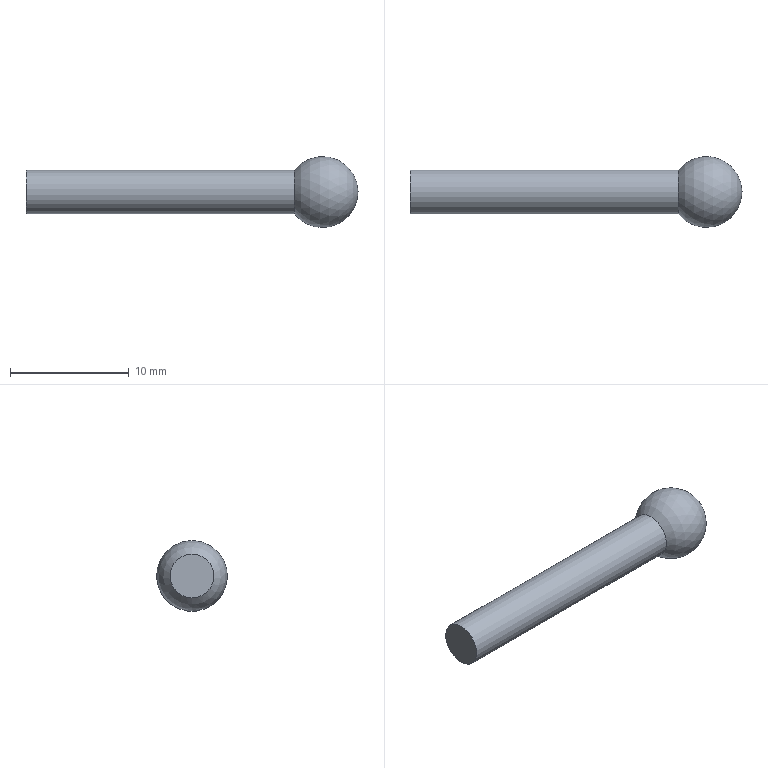Component | NX | CONE_VALVE | 1 solid | 3 faces | box 28 x 6 x 6 mm | volume 353 mm3 | sphere 1 | cylinder 1 | plane 1 | commonest cylinder face diameters 3.7 x1
STEP:
#1=CARTESIAN_POINT('',(0.,0.,0.));
#2=DIRECTION('',(0.,0.,1.));
#3=DIRECTION('',(1.,0.,0.));
#4=AXIS2_PLACEMENT_3D('',#1,#2,#3);
#5=CARTESIAN_POINT('',(-0.5,-0.,18.15));
#6=VERTEX_POINT('',#5);
#7=CARTESIAN_POINT('',(-0.5,-0.,20.));
#8=DIRECTION('',(-1.,0.,0.));
#9=DIRECTION('',(0.,0.,-1.));
#10=AXIS2_PLACEMENT_3D('',#7,#8,#9);
#11=CIRCLE('',#10,1.85);
#12=CARTESIAN_POINT('',(1.862,-0.,20.));
#13=DIRECTION('',(1.,0.,0.));
#14=DIRECTION('',(0.,0.,-1.));
#15=AXIS2_PLACEMENT_3D('',#12,#13,#14);
#16=SPHERICAL_SURFACE('',#15,3.);
#17=CARTESIAN_POINT('',(6.283,-0.9063));
#18=CARTESIAN_POINT('',(6.188,-0.9063));
#19=CARTESIAN_POINT('',(5.998,-0.9063));
#20=CARTESIAN_POINT('',(5.712,-0.9063));
#21=CARTESIAN_POINT('',(5.426,-0.9063));
#22=CARTESIAN_POINT('',(5.141,-0.9063));
#23=CARTESIAN_POINT('',(4.855,-0.9063));
#24=CARTESIAN_POINT('',(4.57,-0.9063));
#25=CARTESIAN_POINT('',(4.284,-0.9063));
#26=CARTESIAN_POINT('',(3.998,-0.9063));
#27=CARTESIAN_POINT('',(3.713,-0.9063));
#28=CARTESIAN_POINT('',(3.427,-0.9063));
#29=CARTESIAN_POINT('',(3.142,-0.9063));
#30=CARTESIAN_POINT('',(2.856,-0.9063));
#31=CARTESIAN_POINT('',(2.57,-0.9063));
#32=CARTESIAN_POINT('',(2.285,-0.9063));
#33=CARTESIAN_POINT('',(1.999,-0.9063));
#34=CARTESIAN_POINT('',(1.714,-0.9063));
#35=CARTESIAN_POINT('',(1.428,-0.9063));
#36=CARTESIAN_POINT('',(1.142,-0.9063));
#37=CARTESIAN_POINT('',(0.8568,-0.9063));
#38=CARTESIAN_POINT('',(0.5712,-0.9063));
#39=CARTESIAN_POINT('',(0.2856,-0.9063));
#40=CARTESIAN_POINT('',(0.0952,-0.9063));
#41=CARTESIAN_POINT('',(0.,-0.9063));
#42=B_SPLINE_CURVE_WITH_KNOTS('',3,(#17,#18,#19,#20,#21,#22,#23,#24,#25,#26,#27,#28,#29,#30,#31,#32,#33,#34,#35,#36,#37,#38,#39,#40,#41),.UNSPECIFIED.,.F.,.F.,(4,1,1,1,1,1,1,1,1,1,1,1,1,1,1,1,1,1,1,1,1,1,4),(0.,0.2856,0.5712,0.8568,1.142,1.428,1.714,1.999,2.285,2.57,2.856,3.142,3.427,3.713,3.998,4.284,4.57,4.855,5.141,5.426,5.712,5.998,6.283),.QUASI_UNIFORM_KNOTS.);
#43=(GEOMETRIC_REPRESENTATION_CONTEXT(2)PARAMETRIC_REPRESENTATION_CONTEXT()REPRESENTATION_CONTEXT('',''));
#44=DEFINITIONAL_REPRESENTATION('',(#42),#43);
#45=PCURVE('',#16,#44);
#46=CARTESIAN_POINT('',(1.862,-0.,20.));
#47=DIRECTION('',(-1.,0.,0.));
#48=DIRECTION('',(0.,0.,1.));
#49=AXIS2_PLACEMENT_3D('',#46,#47,#48);
#50=CYLINDRICAL_SURFACE('',#49,1.85);
#51=CARTESIAN_POINT('',(3.142,2.362));
#52=DIRECTION('',(1.,0.));
#53=VECTOR('',#52,1.);
#54=LINE('',#51,#53);
#55=(GEOMETRIC_REPRESENTATION_CONTEXT(2)PARAMETRIC_REPRESENTATION_CONTEXT()REPRESENTATION_CONTEXT('',''));
#56=DEFINITIONAL_REPRESENTATION('',(#54),#55);
#57=PCURVE('',#50,#56);
#58=SURFACE_CURVE('',#11,(#45,#57),.PCURVE_S1.);
#59=EDGE_CURVE('',#6,#6,#58,.T.);
#60=ORIENTED_EDGE('',*,*,#59,.F.);
#61=CARTESIAN_POINT('',(4.862,-0.,20.));
#62=VERTEX_POINT('',#61);
#63=CARTESIAN_POINT('',(-0.5,-0.,18.15));
#64=CARTESIAN_POINT('',(0.1547,-0.,17.314));
#65=CARTESIAN_POINT('',(1.154,-0.,16.749));
#66=CARTESIAN_POINT('',(2.365,-0.,16.624));
#67=CARTESIAN_POINT('',(3.547,-0.,17.032));
#68=CARTESIAN_POINT('',(4.423,-0.,17.877));
#69=CARTESIAN_POINT('',(4.862,-0.,18.938));
#70=CARTESIAN_POINT('',(4.862,-0.,20.));
#71=B_SPLINE_CURVE_WITH_KNOTS('',7,(#63,#64,#65,#66,#67,#68,#69,#70),.UNSPECIFIED.,.F.,.F.,(8,8),(-0.9063,1.571),.PIECEWISE_BEZIER_KNOTS.);
#72=CARTESIAN_POINT('',(6.283,0.));
#73=DIRECTION('',(0.,1.));
#74=VECTOR('',#73,1.);
#75=LINE('',#72,#74);
#76=(GEOMETRIC_REPRESENTATION_CONTEXT(2)PARAMETRIC_REPRESENTATION_CONTEXT()REPRESENTATION_CONTEXT('',''));
#77=DEFINITIONAL_REPRESENTATION('',(#75),#76);
#78=PCURVE('',#16,#77);
#79=CARTESIAN_POINT('',(0.,0.));
#80=DIRECTION('',(0.,1.));
#81=VECTOR('',#80,1.);
#82=LINE('',#79,#81);
#83=(GEOMETRIC_REPRESENTATION_CONTEXT(2)PARAMETRIC_REPRESENTATION_CONTEXT()REPRESENTATION_CONTEXT('',''));
#84=DEFINITIONAL_REPRESENTATION('',(#82),#83);
#85=PCURVE('',#16,#84);
#86=SEAM_CURVE('',#71,(#78,#85),.PCURVE_S1.);
#87=EDGE_CURVE('',#6,#62,#86,.T.);
#88=ORIENTED_EDGE('',*,*,#87,.T.);
#89=ORIENTED_EDGE('',*,*,#87,.F.);
#90=EDGE_LOOP('',(#60,#88,#89));
#91=FACE_BOUND('',#90,.T.);
#92=ADVANCED_FACE('',(#91),#16,.T.);
#93=ORIENTED_EDGE('',*,*,#59,.T.);
#94=CARTESIAN_POINT('',(-23.138,-0.,18.15));
#95=VERTEX_POINT('',#94);
#96=CARTESIAN_POINT('',(-0.5,-0.,18.15));
#97=CARTESIAN_POINT('',(-23.138,-0.,18.15));
#98=B_SPLINE_CURVE_WITH_KNOTS('',1,(#96,#97),.UNSPECIFIED.,.F.,.F.,(2,2),(2.362,25.),.PIECEWISE_BEZIER_KNOTS.);
#99=CARTESIAN_POINT('',(9.425,0.));
#100=DIRECTION('',(0.,1.));
#101=VECTOR('',#100,1.);
#102=LINE('',#99,#101);
#103=(GEOMETRIC_REPRESENTATION_CONTEXT(2)PARAMETRIC_REPRESENTATION_CONTEXT()REPRESENTATION_CONTEXT('',''));
#104=DEFINITIONAL_REPRESENTATION('',(#102),#103);
#105=PCURVE('',#50,#104);
#106=CARTESIAN_POINT('',(3.142,0.));
#107=DIRECTION('',(0.,1.));
#108=VECTOR('',#107,1.);
#109=LINE('',#106,#108);
#110=(GEOMETRIC_REPRESENTATION_CONTEXT(2)PARAMETRIC_REPRESENTATION_CONTEXT()REPRESENTATION_CONTEXT('',''));
#111=DEFINITIONAL_REPRESENTATION('',(#109),#110);
#112=PCURVE('',#50,#111);
#113=SEAM_CURVE('',#98,(#105,#112),.PCURVE_S1.);
#114=EDGE_CURVE('',#6,#95,#113,.T.);
#115=ORIENTED_EDGE('',*,*,#114,.T.);
#116=CARTESIAN_POINT('',(-23.138,-0.,20.));
#117=DIRECTION('',(1.,0.,0.));
#118=DIRECTION('',(0.,0.,-1.));
#119=AXIS2_PLACEMENT_3D('',#116,#117,#118);
#120=CIRCLE('',#119,1.85);
#121=CARTESIAN_POINT('',(9.425,25.));
#122=DIRECTION('',(-1.,0.));
#123=VECTOR('',#122,1.);
#124=LINE('',#121,#123);
#125=(GEOMETRIC_REPRESENTATION_CONTEXT(2)PARAMETRIC_REPRESENTATION_CONTEXT()REPRESENTATION_CONTEXT('',''));
#126=DEFINITIONAL_REPRESENTATION('',(#124),#125);
#127=PCURVE('',#50,#126);
#128=CARTESIAN_POINT('',(-23.138,-0.,20.));
#129=DIRECTION('',(1.,0.,0.));
#130=DIRECTION('',(0.,0.,-1.));
#131=AXIS2_PLACEMENT_3D('',#128,#129,#130);
#132=PLANE('',#131);
#133=CARTESIAN_POINT('',(0.,0.));
#134=DIRECTION('',(1.,0.));
#135=AXIS2_PLACEMENT_2D('',#133,#134);
#136=CIRCLE('',#135,1.85);
#137=(GEOMETRIC_REPRESENTATION_CONTEXT(2)PARAMETRIC_REPRESENTATION_CONTEXT()REPRESENTATION_CONTEXT('',''));
#138=DEFINITIONAL_REPRESENTATION('',(#136),#137);
#139=PCURVE('',#132,#138);
#140=SURFACE_CURVE('',#120,(#127,#139),.PCURVE_S1.);
#141=EDGE_CURVE('',#95,#95,#140,.T.);
#142=ORIENTED_EDGE('',*,*,#141,.T.);
#143=ORIENTED_EDGE('',*,*,#114,.F.);
#144=EDGE_LOOP('',(#93,#115,#142,#143));
#145=FACE_BOUND('',#144,.T.);
#146=ADVANCED_FACE('',(#145),#50,.T.);
#147=ORIENTED_EDGE('',*,*,#141,.F.);
#148=EDGE_LOOP('',(#147));
#149=FACE_BOUND('',#148,.T.);
#150=ADVANCED_FACE('',(#149),#132,.F.);
#151=CLOSED_SHELL('',(#92,#146,#150));
#152=MANIFOLD_SOLID_BREP('',#151);
#153=(LENGTH_UNIT()NAMED_UNIT(*)SI_UNIT(.MILLI.,.METRE.));
#154=UNCERTAINTY_MEASURE_WITH_UNIT(LENGTH_MEASURE(0.00001),#153,'','');
#155=(NAMED_UNIT(*)PLANE_ANGLE_UNIT()SI_UNIT($,.RADIAN.));
#156=(NAMED_UNIT(*)SI_UNIT($,.STERADIAN.)SOLID_ANGLE_UNIT());
#157=(GEOMETRIC_REPRESENTATION_CONTEXT(3)GLOBAL_UNCERTAINTY_ASSIGNED_CONTEXT((#154))GLOBAL_UNIT_ASSIGNED_CONTEXT((#153,#155,#156))REPRESENTATION_CONTEXT('',''));
#158=ADVANCED_BREP_SHAPE_REPRESENTATION('',(#4,#152),#157);